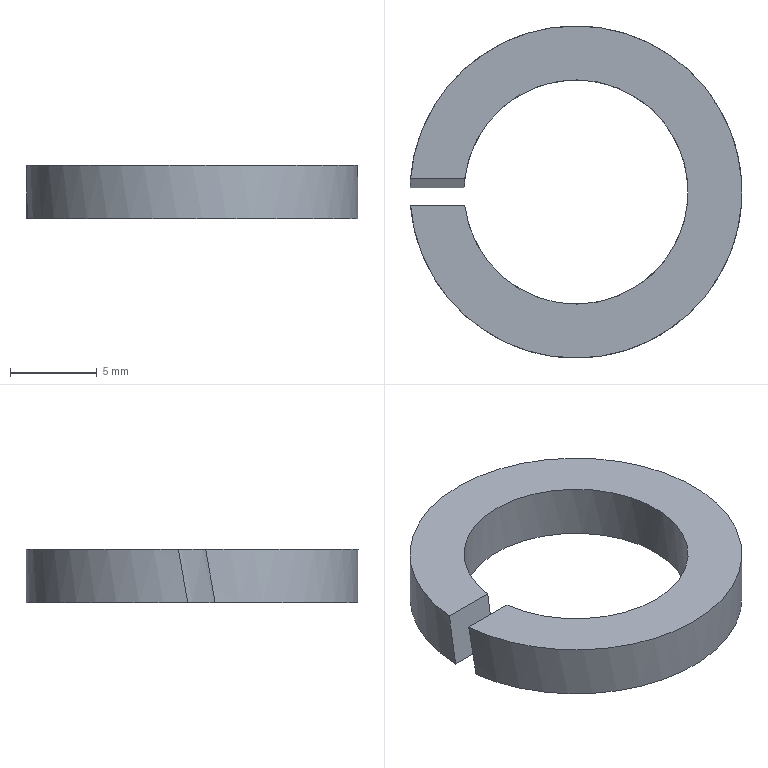Component | NX | GB93-87_12_11 | 1 solid | 6 faces | box 19.1 x 19.1 x 3.1 mm | volume 468 mm3 | plane 4 | cylinder 2 | commonest cylinder face diameters 19.1 x1 12.9 x1
STEP:
#1=CARTESIAN_POINT('',(0.,0.,0.));
#2=DIRECTION('',(0.,0.,1.));
#3=DIRECTION('',(1.,0.,0.));
#4=AXIS2_PLACEMENT_3D('',#1,#2,#3);
#5=CARTESIAN_POINT('',(-104.518,138.213,-118.));
#6=VERTEX_POINT('',#5);
#7=CARTESIAN_POINT('',(-104.518,139.787,-118.));
#8=VERTEX_POINT('',#7);
#9=CARTESIAN_POINT('',(-95.,139.,-118.));
#10=DIRECTION('',(0.,0.,1.));
#11=DIRECTION('',(1.,0.,0.));
#12=AXIS2_PLACEMENT_3D('',#9,#10,#11);
#13=CIRCLE('',#12,9.55);
#14=CARTESIAN_POINT('',(-95.,139.,-118.));
#15=DIRECTION('',(0.,0.,1.));
#16=DIRECTION('',(1.,0.,0.));
#17=AXIS2_PLACEMENT_3D('',#14,#15,#16);
#18=CYLINDRICAL_SURFACE('',#17,9.55);
#19=CARTESIAN_POINT('',(-6.283,0.));
#20=DIRECTION('',(1.,0.));
#21=VECTOR('',#20,1.);
#22=LINE('',#19,#21);
#23=(GEOMETRIC_REPRESENTATION_CONTEXT(2)PARAMETRIC_REPRESENTATION_CONTEXT()REPRESENTATION_CONTEXT('',''));
#24=DEFINITIONAL_REPRESENTATION('',(#22),#23);
#25=PCURVE('',#18,#24);
#26=CARTESIAN_POINT('',(-95.,145.45,-118.));
#27=DIRECTION('',(0.,0.,1.));
#28=DIRECTION('',(1.,0.,0.));
#29=AXIS2_PLACEMENT_3D('',#26,#27,#28);
#30=PLANE('',#29);
#31=CARTESIAN_POINT('',(0.,-6.45));
#32=DIRECTION('',(1.,0.));
#33=AXIS2_PLACEMENT_2D('',#31,#32);
#34=CIRCLE('',#33,9.55);
#35=(GEOMETRIC_REPRESENTATION_CONTEXT(2)PARAMETRIC_REPRESENTATION_CONTEXT()REPRESENTATION_CONTEXT('',''));
#36=DEFINITIONAL_REPRESENTATION('',(#34),#35);
#37=PCURVE('',#30,#36);
#38=SURFACE_CURVE('',#13,(#25,#37),.PCURVE_S1.);
#39=EDGE_CURVE('',#6,#8,#38,.T.);
#40=ORIENTED_EDGE('',*,*,#39,.F.);
#41=CARTESIAN_POINT('',(-104.456,137.666,-121.1));
#42=VERTEX_POINT('',#41);
#43=CARTESIAN_POINT('',(-95.,139.,-113.537));
#44=DIRECTION('',(0.,-0.9848,0.1736));
#45=DIRECTION('',(0.,0.1736,0.9848));
#46=AXIS2_PLACEMENT_3D('',#43,#44,#45);
#47=ELLIPSE('',#46,54.996,9.55);
#48=CARTESIAN_POINT('',(-3.059,0.));
#49=CARTESIAN_POINT('',(-3.001,-3.1));
#50=B_SPLINE_CURVE_WITH_KNOTS('',1,(#48,#49),.UNSPECIFIED.,.F.,.F.,(2,2),(1.653,1.711),.PIECEWISE_BEZIER_KNOTS.);
#51=(GEOMETRIC_REPRESENTATION_CONTEXT(2)PARAMETRIC_REPRESENTATION_CONTEXT()REPRESENTATION_CONTEXT('',''));
#52=DEFINITIONAL_REPRESENTATION('',(#50),#51);
#53=PCURVE('',#18,#52);
#54=CARTESIAN_POINT('',(-109.325,137.429,-122.445));
#55=DIRECTION('',(0.,0.9848,-0.1736));
#56=DIRECTION('',(0.,-0.1736,-0.9848));
#57=AXIS2_PLACEMENT_3D('',#54,#55,#56);
#58=PLANE('',#57);
#59=CARTESIAN_POINT('',(-64.042,-14.325));
#60=CARTESIAN_POINT('',(-64.042,2.216));
#61=CARTESIAN_POINT('',(18.453,-6.054));
#62=CARTESIAN_POINT('',(100.947,-14.325));
#63=CARTESIAN_POINT('',(18.453,-22.596));
#64=CARTESIAN_POINT('',(-64.042,-30.866));
#65=CARTESIAN_POINT('',(-64.042,-14.325));
#66=(BOUNDED_CURVE()B_SPLINE_CURVE(2,(#59,#60,#61,#62,#63,#64,#65),.UNSPECIFIED.,.T.,.F.)B_SPLINE_CURVE_WITH_KNOTS((1,2,2,2,2,1),(-2.094,0.,2.094,4.189,6.283,8.378),.UNSPECIFIED.)CURVE()GEOMETRIC_REPRESENTATION_ITEM()RATIONAL_B_SPLINE_CURVE((1.,0.5,1.,0.5,1.,0.5,1.))REPRESENTATION_ITEM(''));
#67=(GEOMETRIC_REPRESENTATION_CONTEXT(2)PARAMETRIC_REPRESENTATION_CONTEXT()REPRESENTATION_CONTEXT('',''));
#68=DEFINITIONAL_REPRESENTATION('',(#66),#67);
#69=PCURVE('',#58,#68);
#70=SURFACE_CURVE('',#47,(#53,#69),.PCURVE_S1.);
#71=EDGE_CURVE('',#6,#42,#70,.T.);
#72=ORIENTED_EDGE('',*,*,#71,.T.);
#73=CARTESIAN_POINT('',(-104.547,139.24,-121.1));
#74=VERTEX_POINT('',#73);
#75=CARTESIAN_POINT('',(-95.,139.,-121.1));
#76=DIRECTION('',(0.,0.,1.));
#77=DIRECTION('',(1.,0.,0.));
#78=AXIS2_PLACEMENT_3D('',#75,#76,#77);
#79=CIRCLE('',#78,9.55);
#80=CARTESIAN_POINT('',(-6.283,-3.1));
#81=DIRECTION('',(1.,0.));
#82=VECTOR('',#81,1.);
#83=LINE('',#80,#82);
#84=(GEOMETRIC_REPRESENTATION_CONTEXT(2)PARAMETRIC_REPRESENTATION_CONTEXT()REPRESENTATION_CONTEXT('',''));
#85=DEFINITIONAL_REPRESENTATION('',(#83),#84);
#86=PCURVE('',#18,#85);
#87=CARTESIAN_POINT('',(-95.,148.55,-121.1));
#88=DIRECTION('',(0.,0.,-1.));
#89=DIRECTION('',(-1.,0.,0.));
#90=AXIS2_PLACEMENT_3D('',#87,#88,#89);
#91=PLANE('',#90);
#92=CARTESIAN_POINT('',(-9.55,-9.55));
#93=CARTESIAN_POINT('',(-9.55,6.991));
#94=CARTESIAN_POINT('',(4.775,-1.279));
#95=CARTESIAN_POINT('',(19.1,-9.55));
#96=CARTESIAN_POINT('',(4.775,-17.821));
#97=CARTESIAN_POINT('',(-9.55,-26.091));
#98=CARTESIAN_POINT('',(-9.55,-9.55));
#99=(BOUNDED_CURVE()B_SPLINE_CURVE(2,(#92,#93,#94,#95,#96,#97,#98),.UNSPECIFIED.,.T.,.F.)B_SPLINE_CURVE_WITH_KNOTS((1,2,2,2,2,1),(-2.094,0.,2.094,4.189,6.283,8.378),.UNSPECIFIED.)CURVE()GEOMETRIC_REPRESENTATION_ITEM()RATIONAL_B_SPLINE_CURVE((1.,0.5,1.,0.5,1.,0.5,1.))REPRESENTATION_ITEM(''));
#100=(GEOMETRIC_REPRESENTATION_CONTEXT(2)PARAMETRIC_REPRESENTATION_CONTEXT()REPRESENTATION_CONTEXT('',''));
#101=DEFINITIONAL_REPRESENTATION('',(#99),#100);
#102=PCURVE('',#91,#101);
#103=SURFACE_CURVE('',#79,(#86,#102),.PCURVE_S1.);
#104=EDGE_CURVE('',#42,#74,#103,.T.);
#105=ORIENTED_EDGE('',*,*,#104,.T.);
#106=CARTESIAN_POINT('',(-95.,139.,-122.463));
#107=DIRECTION('',(0.,0.9848,-0.1736));
#108=DIRECTION('',(0.,0.1736,0.9848));
#109=AXIS2_PLACEMENT_3D('',#106,#107,#108);
#110=ELLIPSE('',#109,54.996,9.55);
#111=CARTESIAN_POINT('',(3.116,-3.1));
#112=CARTESIAN_POINT('',(3.059,-0.));
#113=B_SPLINE_CURVE_WITH_KNOTS('',1,(#111,#112),.UNSPECIFIED.,.F.,.F.,(2,2),(4.738,4.795),.PIECEWISE_BEZIER_KNOTS.);
#114=(GEOMETRIC_REPRESENTATION_CONTEXT(2)PARAMETRIC_REPRESENTATION_CONTEXT()REPRESENTATION_CONTEXT('',''));
#115=DEFINITIONAL_REPRESENTATION('',(#113),#114);
#116=PCURVE('',#18,#115);
#117=CARTESIAN_POINT('',(-109.325,140.571,-113.555));
#118=DIRECTION('',(0.,-0.9848,0.1736));
#119=DIRECTION('',(0.,0.1736,0.9848));
#120=AXIS2_PLACEMENT_3D('',#117,#118,#119);
#121=PLANE('',#120);
#122=CARTESIAN_POINT('',(45.951,-14.325));
#123=CARTESIAN_POINT('',(45.951,-30.866));
#124=CARTESIAN_POINT('',(-36.543,-22.596));
#125=CARTESIAN_POINT('',(-119.038,-14.325));
#126=CARTESIAN_POINT('',(-36.543,-6.054));
#127=CARTESIAN_POINT('',(45.951,2.216));
#128=CARTESIAN_POINT('',(45.951,-14.325));
#129=(BOUNDED_CURVE()B_SPLINE_CURVE(2,(#122,#123,#124,#125,#126,#127,#128),.UNSPECIFIED.,.T.,.F.)B_SPLINE_CURVE_WITH_KNOTS((1,2,2,2,2,1),(-2.094,0.,2.094,4.189,6.283,8.378),.UNSPECIFIED.)CURVE()GEOMETRIC_REPRESENTATION_ITEM()RATIONAL_B_SPLINE_CURVE((1.,0.5,1.,0.5,1.,0.5,1.))REPRESENTATION_ITEM(''));
#130=(GEOMETRIC_REPRESENTATION_CONTEXT(2)PARAMETRIC_REPRESENTATION_CONTEXT()REPRESENTATION_CONTEXT('',''));
#131=DEFINITIONAL_REPRESENTATION('',(#129),#130);
#132=PCURVE('',#121,#131);
#133=SURFACE_CURVE('',#110,(#116,#132),.PCURVE_S1.);
#134=EDGE_CURVE('',#74,#8,#133,.T.);
#135=ORIENTED_EDGE('',*,*,#134,.T.);
#136=EDGE_LOOP('',(#40,#72,#105,#135));
#137=FACE_BOUND('',#136,.T.);
#138=ADVANCED_FACE('',(#137),#18,.T.);
#139=ORIENTED_EDGE('',*,*,#104,.F.);
#140=CARTESIAN_POINT('',(-101.311,137.666,-121.1));
#141=VERTEX_POINT('',#140);
#142=CARTESIAN_POINT('',(-95.,137.666,-121.1));
#143=DIRECTION('',(1.,0.,0.));
#144=VECTOR('',#143,1.);
#145=LINE('',#142,#144);
#146=CARTESIAN_POINT('',(0.,-10.884));
#147=DIRECTION('',(-1.,0.));
#148=VECTOR('',#147,1.);
#149=LINE('',#146,#148);
#150=(GEOMETRIC_REPRESENTATION_CONTEXT(2)PARAMETRIC_REPRESENTATION_CONTEXT()REPRESENTATION_CONTEXT('',''));
#151=DEFINITIONAL_REPRESENTATION('',(#149),#150);
#152=PCURVE('',#91,#151);
#153=CARTESIAN_POINT('',(-1.366,-14.325));
#154=DIRECTION('',(0.,-1.));
#155=VECTOR('',#154,1.);
#156=LINE('',#153,#155);
#157=(GEOMETRIC_REPRESENTATION_CONTEXT(2)PARAMETRIC_REPRESENTATION_CONTEXT()REPRESENTATION_CONTEXT('',''));
#158=DEFINITIONAL_REPRESENTATION('',(#156),#157);
#159=PCURVE('',#58,#158);
#160=SURFACE_CURVE('',#145,(#152,#159),.PCURVE_S1.);
#161=EDGE_CURVE('',#42,#141,#160,.T.);
#162=ORIENTED_EDGE('',*,*,#161,.T.);
#163=CARTESIAN_POINT('',(-101.446,139.24,-121.1));
#164=VERTEX_POINT('',#163);
#165=CARTESIAN_POINT('',(-95.,139.,-121.1));
#166=DIRECTION('',(0.,0.,1.));
#167=DIRECTION('',(1.,0.,0.));
#168=AXIS2_PLACEMENT_3D('',#165,#166,#167);
#169=CIRCLE('',#168,6.45);
#170=CARTESIAN_POINT('',(-6.45,-9.55));
#171=CARTESIAN_POINT('',(-6.45,1.622));
#172=CARTESIAN_POINT('',(3.225,-3.964));
#173=CARTESIAN_POINT('',(12.9,-9.55));
#174=CARTESIAN_POINT('',(3.225,-15.136));
#175=CARTESIAN_POINT('',(-6.45,-20.722));
#176=CARTESIAN_POINT('',(-6.45,-9.55));
#177=(BOUNDED_CURVE()B_SPLINE_CURVE(2,(#170,#171,#172,#173,#174,#175,#176),.UNSPECIFIED.,.T.,.F.)B_SPLINE_CURVE_WITH_KNOTS((1,2,2,2,2,1),(-2.094,0.,2.094,4.189,6.283,8.378),.UNSPECIFIED.)CURVE()GEOMETRIC_REPRESENTATION_ITEM()RATIONAL_B_SPLINE_CURVE((1.,0.5,1.,0.5,1.,0.5,1.))REPRESENTATION_ITEM(''));
#178=(GEOMETRIC_REPRESENTATION_CONTEXT(2)PARAMETRIC_REPRESENTATION_CONTEXT()REPRESENTATION_CONTEXT('',''));
#179=DEFINITIONAL_REPRESENTATION('',(#177),#178);
#180=PCURVE('',#91,#179);
#181=CARTESIAN_POINT('',(-95.,139.,-118.));
#182=DIRECTION('',(0.,0.,1.));
#183=DIRECTION('',(1.,0.,0.));
#184=AXIS2_PLACEMENT_3D('',#181,#182,#183);
#185=CYLINDRICAL_SURFACE('',#184,6.45);
#186=CARTESIAN_POINT('',(-6.283,-3.1));
#187=DIRECTION('',(1.,0.));
#188=VECTOR('',#187,1.);
#189=LINE('',#186,#188);
#190=(GEOMETRIC_REPRESENTATION_CONTEXT(2)PARAMETRIC_REPRESENTATION_CONTEXT()REPRESENTATION_CONTEXT('',''));
#191=DEFINITIONAL_REPRESENTATION('',(#189),#190);
#192=PCURVE('',#185,#191);
#193=SURFACE_CURVE('',#169,(#180,#192),.PCURVE_S1.);
#194=EDGE_CURVE('',#141,#164,#193,.T.);
#195=ORIENTED_EDGE('',*,*,#194,.T.);
#196=CARTESIAN_POINT('',(-95.,139.24,-121.1));
#197=DIRECTION('',(-1.,0.,0.));
#198=VECTOR('',#197,1.);
#199=LINE('',#196,#198);
#200=CARTESIAN_POINT('',(0.,-9.31));
#201=DIRECTION('',(1.,0.));
#202=VECTOR('',#201,1.);
#203=LINE('',#200,#202);
#204=(GEOMETRIC_REPRESENTATION_CONTEXT(2)PARAMETRIC_REPRESENTATION_CONTEXT()REPRESENTATION_CONTEXT('',''));
#205=DEFINITIONAL_REPRESENTATION('',(#203),#204);
#206=PCURVE('',#91,#205);
#207=CARTESIAN_POINT('',(-7.661,-14.325));
#208=DIRECTION('',(0.,1.));
#209=VECTOR('',#208,1.);
#210=LINE('',#207,#209);
#211=(GEOMETRIC_REPRESENTATION_CONTEXT(2)PARAMETRIC_REPRESENTATION_CONTEXT()REPRESENTATION_CONTEXT('',''));
#212=DEFINITIONAL_REPRESENTATION('',(#210),#211);
#213=PCURVE('',#121,#212);
#214=SURFACE_CURVE('',#199,(#206,#213),.PCURVE_S1.);
#215=EDGE_CURVE('',#164,#74,#214,.T.);
#216=ORIENTED_EDGE('',*,*,#215,.T.);
#217=EDGE_LOOP('',(#139,#162,#195,#216));
#218=FACE_BOUND('',#217,.T.);
#219=ADVANCED_FACE('',(#218),#91,.T.);
#220=CARTESIAN_POINT('',(-101.402,139.787,-118.));
#221=VERTEX_POINT('',#220);
#222=CARTESIAN_POINT('',(-95.,139.,-122.463));
#223=DIRECTION('',(0.,-0.9848,0.1736));
#224=DIRECTION('',(0.,0.1736,0.9848));
#225=AXIS2_PLACEMENT_3D('',#222,#223,#224);
#226=ELLIPSE('',#225,37.144,6.45);
#227=CARTESIAN_POINT('',(3.019,-0.));
#228=CARTESIAN_POINT('',(3.104,-3.1));
#229=B_SPLINE_CURVE_WITH_KNOTS('',1,(#227,#228),.UNSPECIFIED.,.F.,.F.,(2,2),(1.448,1.534),.PIECEWISE_BEZIER_KNOTS.);
#230=(GEOMETRIC_REPRESENTATION_CONTEXT(2)PARAMETRIC_REPRESENTATION_CONTEXT()REPRESENTATION_CONTEXT('',''));
#231=DEFINITIONAL_REPRESENTATION('',(#229),#230);
#232=PCURVE('',#185,#231);
#233=CARTESIAN_POINT('',(-9.045,-14.325));
#234=DIRECTION('',(1.,0.));
#235=AXIS2_PLACEMENT_2D('',#233,#234);
#236=ELLIPSE('',#235,37.144,6.45);
#237=(GEOMETRIC_REPRESENTATION_CONTEXT(2)PARAMETRIC_REPRESENTATION_CONTEXT()REPRESENTATION_CONTEXT('',''));
#238=DEFINITIONAL_REPRESENTATION('',(#236),#237);
#239=PCURVE('',#121,#238);
#240=SURFACE_CURVE('',#226,(#232,#239),.PCURVE_S1.);
#241=EDGE_CURVE('',#221,#164,#240,.T.);
#242=ORIENTED_EDGE('',*,*,#241,.F.);
#243=CARTESIAN_POINT('',(-101.402,138.213,-118.));
#244=VERTEX_POINT('',#243);
#245=CARTESIAN_POINT('',(-95.,139.,-118.));
#246=DIRECTION('',(0.,0.,1.));
#247=DIRECTION('',(1.,0.,0.));
#248=AXIS2_PLACEMENT_3D('',#245,#246,#247);
#249=CIRCLE('',#248,6.45);
#250=CARTESIAN_POINT('',(-6.283,0.));
#251=DIRECTION('',(1.,0.));
#252=VECTOR('',#251,1.);
#253=LINE('',#250,#252);
#254=(GEOMETRIC_REPRESENTATION_CONTEXT(2)PARAMETRIC_REPRESENTATION_CONTEXT()REPRESENTATION_CONTEXT('',''));
#255=DEFINITIONAL_REPRESENTATION('',(#253),#254);
#256=PCURVE('',#185,#255);
#257=CARTESIAN_POINT('',(0.,-6.45));
#258=DIRECTION('',(1.,0.));
#259=AXIS2_PLACEMENT_2D('',#257,#258);
#260=CIRCLE('',#259,6.45);
#261=(GEOMETRIC_REPRESENTATION_CONTEXT(2)PARAMETRIC_REPRESENTATION_CONTEXT()REPRESENTATION_CONTEXT('',''));
#262=DEFINITIONAL_REPRESENTATION('',(#260),#261);
#263=PCURVE('',#30,#262);
#264=SURFACE_CURVE('',#249,(#256,#263),.PCURVE_S1.);
#265=EDGE_CURVE('',#244,#221,#264,.T.);
#266=ORIENTED_EDGE('',*,*,#265,.F.);
#267=CARTESIAN_POINT('',(-95.,139.,-113.537));
#268=DIRECTION('',(0.,0.9848,-0.1736));
#269=DIRECTION('',(0.,0.1736,0.9848));
#270=AXIS2_PLACEMENT_3D('',#267,#268,#269);
#271=ELLIPSE('',#270,37.144,6.45);
#272=CARTESIAN_POINT('',(-2.933,-3.1));
#273=CARTESIAN_POINT('',(-3.019,0.));
#274=B_SPLINE_CURVE_WITH_KNOTS('',1,(#272,#273),.UNSPECIFIED.,.F.,.F.,(2,2),(4.504,4.59),.PIECEWISE_BEZIER_KNOTS.);
#275=(GEOMETRIC_REPRESENTATION_CONTEXT(2)PARAMETRIC_REPRESENTATION_CONTEXT()REPRESENTATION_CONTEXT('',''));
#276=DEFINITIONAL_REPRESENTATION('',(#274),#275);
#277=PCURVE('',#185,#276);
#278=CARTESIAN_POINT('',(-9.045,-14.325));
#279=DIRECTION('',(-1.,0.));
#280=AXIS2_PLACEMENT_2D('',#278,#279);
#281=ELLIPSE('',#280,37.144,6.45);
#282=(GEOMETRIC_REPRESENTATION_CONTEXT(2)PARAMETRIC_REPRESENTATION_CONTEXT()REPRESENTATION_CONTEXT('',''));
#283=DEFINITIONAL_REPRESENTATION('',(#281),#282);
#284=PCURVE('',#58,#283);
#285=SURFACE_CURVE('',#271,(#277,#284),.PCURVE_S1.);
#286=EDGE_CURVE('',#141,#244,#285,.T.);
#287=ORIENTED_EDGE('',*,*,#286,.F.);
#288=ORIENTED_EDGE('',*,*,#194,.T.);
#289=EDGE_LOOP('',(#242,#266,#287,#288));
#290=FACE_BOUND('',#289,.F.);
#291=ADVANCED_FACE('',(#290),#185,.F.);
#292=ORIENTED_EDGE('',*,*,#265,.F.);
#293=CARTESIAN_POINT('',(-95.,138.213,-118.));
#294=DIRECTION('',(-1.,0.,0.));
#295=VECTOR('',#294,1.);
#296=LINE('',#293,#295);
#297=CARTESIAN_POINT('',(0.,-7.237));
#298=DIRECTION('',(-1.,0.));
#299=VECTOR('',#298,1.);
#300=LINE('',#297,#299);
#301=(GEOMETRIC_REPRESENTATION_CONTEXT(2)PARAMETRIC_REPRESENTATION_CONTEXT()REPRESENTATION_CONTEXT('',''));
#302=DEFINITIONAL_REPRESENTATION('',(#300),#301);
#303=PCURVE('',#30,#302);
#304=CARTESIAN_POINT('',(-4.513,-14.325));
#305=DIRECTION('',(0.,1.));
#306=VECTOR('',#305,1.);
#307=LINE('',#304,#306);
#308=(GEOMETRIC_REPRESENTATION_CONTEXT(2)PARAMETRIC_REPRESENTATION_CONTEXT()REPRESENTATION_CONTEXT('',''));
#309=DEFINITIONAL_REPRESENTATION('',(#307),#308);
#310=PCURVE('',#58,#309);
#311=SURFACE_CURVE('',#296,(#303,#310),.PCURVE_S1.);
#312=EDGE_CURVE('',#244,#6,#311,.T.);
#313=ORIENTED_EDGE('',*,*,#312,.T.);
#314=ORIENTED_EDGE('',*,*,#39,.T.);
#315=CARTESIAN_POINT('',(-95.,139.787,-118.));
#316=DIRECTION('',(1.,0.,0.));
#317=VECTOR('',#316,1.);
#318=LINE('',#315,#317);
#319=CARTESIAN_POINT('',(0.,-5.663));
#320=DIRECTION('',(1.,0.));
#321=VECTOR('',#320,1.);
#322=LINE('',#319,#321);
#323=(GEOMETRIC_REPRESENTATION_CONTEXT(2)PARAMETRIC_REPRESENTATION_CONTEXT()REPRESENTATION_CONTEXT('',''));
#324=DEFINITIONAL_REPRESENTATION('',(#322),#323);
#325=PCURVE('',#30,#324);
#326=CARTESIAN_POINT('',(-4.513,-14.325));
#327=DIRECTION('',(0.,-1.));
#328=VECTOR('',#327,1.);
#329=LINE('',#326,#328);
#330=(GEOMETRIC_REPRESENTATION_CONTEXT(2)PARAMETRIC_REPRESENTATION_CONTEXT()REPRESENTATION_CONTEXT('',''));
#331=DEFINITIONAL_REPRESENTATION('',(#329),#330);
#332=PCURVE('',#121,#331);
#333=SURFACE_CURVE('',#318,(#325,#332),.PCURVE_S1.);
#334=EDGE_CURVE('',#8,#221,#333,.T.);
#335=ORIENTED_EDGE('',*,*,#334,.T.);
#336=EDGE_LOOP('',(#292,#313,#314,#335));
#337=FACE_BOUND('',#336,.T.);
#338=ADVANCED_FACE('',(#337),#30,.T.);
#339=ORIENTED_EDGE('',*,*,#215,.F.);
#340=ORIENTED_EDGE('',*,*,#241,.F.);
#341=ORIENTED_EDGE('',*,*,#334,.F.);
#342=ORIENTED_EDGE('',*,*,#134,.F.);
#343=EDGE_LOOP('',(#339,#340,#341,#342));
#344=FACE_BOUND('',#343,.T.);
#345=ADVANCED_FACE('',(#344),#121,.T.);
#346=ORIENTED_EDGE('',*,*,#312,.F.);
#347=ORIENTED_EDGE('',*,*,#286,.F.);
#348=ORIENTED_EDGE('',*,*,#161,.F.);
#349=ORIENTED_EDGE('',*,*,#71,.F.);
#350=EDGE_LOOP('',(#346,#347,#348,#349));
#351=FACE_BOUND('',#350,.T.);
#352=ADVANCED_FACE('',(#351),#58,.T.);
#353=CLOSED_SHELL('',(#138,#219,#291,#338,#345,#352));
#354=MANIFOLD_SOLID_BREP('',#353);
#355=(LENGTH_UNIT()NAMED_UNIT(*)SI_UNIT(.MILLI.,.METRE.));
#356=UNCERTAINTY_MEASURE_WITH_UNIT(LENGTH_MEASURE(0.002),#355,'','');
#357=(NAMED_UNIT(*)PLANE_ANGLE_UNIT()SI_UNIT($,.RADIAN.));
#358=(NAMED_UNIT(*)SI_UNIT($,.STERADIAN.)SOLID_ANGLE_UNIT());
#359=(GEOMETRIC_REPRESENTATION_CONTEXT(3)GLOBAL_UNCERTAINTY_ASSIGNED_CONTEXT((#356))GLOBAL_UNIT_ASSIGNED_CONTEXT((#355,#357,#358))REPRESENTATION_CONTEXT('',''));
#360=ADVANCED_BREP_SHAPE_REPRESENTATION('',(#4,#354),#359);